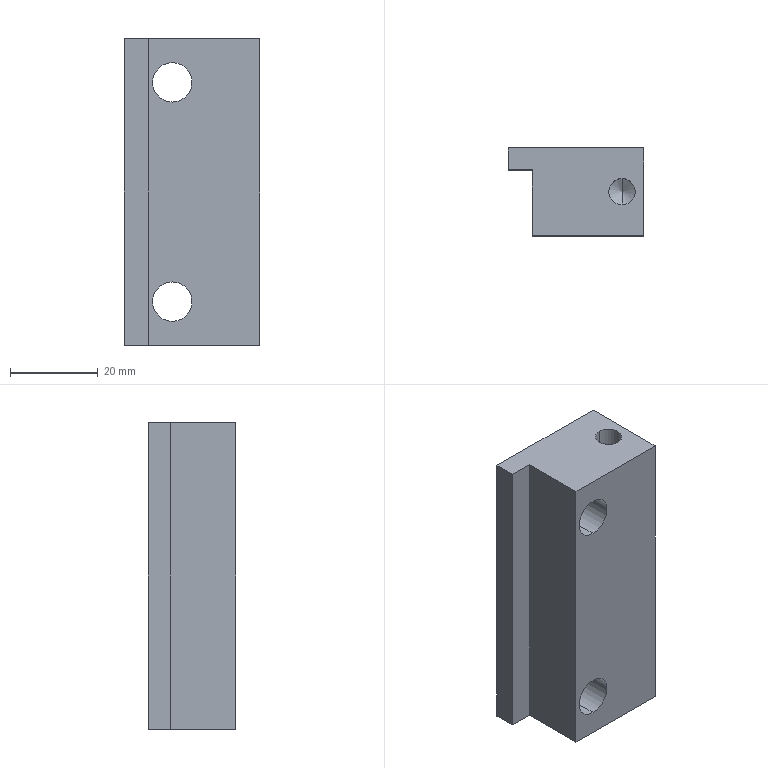Component | SolidWorks | CTM-T-12-AG-05-1 | 1 solid | 20 faces | box 31 x 20 x 70 mm | volume 34085 mm3 | cylinder 8 | plane 8 | cone 4 | commonest cylinder face diameters 9 x4 6 x4 | material Q235A
build123d program:
from build123d import *

# Parameters (mm, degrees)
BOSS_EXTRUDE1_DEPTH      = 70
M6_TAPPED_HOLE1_D        = 6
M6_TAPPED_HOLE1_DEPTH    = 17
M6_TAPPED_HOLE1_TIP      = 1.803
M6_TAPPED_HOLE2_D        = 6
M6_TAPPED_HOLE2_DEPTH    = 17
M6_TAPPED_HOLE2_TIP      = 1.803
M8_CLEARANCE_HOLE1_D     = 9
M8_CLEARANCE_HOLE1_DEPTH = 20
M8_CLEARANCE_HOLE1_TIP   = 2.704


with BuildPart() as part:
    # Sketch1 → Boss-Extrude1 (new body)
    with BuildSketch(Plane.XY):
        Polygon((5, 31), (5, 25.5), (20, 25.5), (20, 0), (0, 0), (0, 31), align=None)
    extrude(amount=BOSS_EXTRUDE1_DEPTH)

    # M6 Tapped Hole1
    with Locations(Plane(origin=(0, 0, 0), x_dir=(-1, 0, 0), z_dir=(0, 0, -1))):
        with Locations((-10, 5)):
            Hole(M6_TAPPED_HOLE1_D / 2, depth=M6_TAPPED_HOLE1_DEPTH)
            with Locations((0, 0, -(M6_TAPPED_HOLE1_DEPTH + M6_TAPPED_HOLE1_TIP / 2))):  # 118° drill point
                Cone(0, M6_TAPPED_HOLE1_D / 2, M6_TAPPED_HOLE1_TIP, mode=Mode.SUBTRACT)

    # M6 Tapped Hole2
    with Locations(Plane.XY.offset(70)):
        with Locations((10, 5)):
            Hole(M6_TAPPED_HOLE2_D / 2, depth=M6_TAPPED_HOLE2_DEPTH)
            with Locations((0, 0, -(M6_TAPPED_HOLE2_DEPTH + M6_TAPPED_HOLE2_TIP / 2))):  # 118° drill point
                Cone(0, M6_TAPPED_HOLE2_D / 2, M6_TAPPED_HOLE2_TIP, mode=Mode.SUBTRACT)

    # M8 Clearance Hole1
    with Locations(Plane.ZY):
        with Locations((10, 20), (60, 20)):
            Hole(M8_CLEARANCE_HOLE1_D / 2, depth=M8_CLEARANCE_HOLE1_DEPTH)
            with Locations((0, 0, -(M8_CLEARANCE_HOLE1_DEPTH + M8_CLEARANCE_HOLE1_TIP / 2))):  # 118° drill point
                Cone(0, M8_CLEARANCE_HOLE1_D / 2, M8_CLEARANCE_HOLE1_TIP, mode=Mode.SUBTRACT)


solid = part.part

# Placed as in the assembly
solid = solid.moved(Location((90.4, 0, 70), (180, 0, 90)))
STEP:
#1=CARTESIAN_POINT('',(2.772,-0.7874,2.539));
#2=VERTEX_POINT('',#1);
#3=CARTESIAN_POINT('',(2.772,-0.7874,2.185));
#4=VERTEX_POINT('',#3);
#5=CARTESIAN_POINT('',(2.772,-0.7874,2.362));
#6=DIRECTION('',(0.,1.,0.));
#7=DIRECTION('',(0.,0.,-1.));
#8=AXIS2_PLACEMENT_3D('',#5,#6,#7);
#9=CIRCLE('',#8,0.1772);
#10=EDGE_CURVE('',#2,#4,#9,.T.);
#11=ORIENTED_EDGE('',*,*,#10,.F.);
#12=CARTESIAN_POINT('',(2.772,0.,2.539));
#13=VERTEX_POINT('',#12);
#14=CARTESIAN_POINT('',(2.772,0.,2.539));
#15=DIRECTION('',(0.,1.,0.));
#16=VECTOR('',#15,39.37);
#17=LINE('',#14,#16);
#18=EDGE_CURVE('',#2,#13,#17,.T.);
#19=ORIENTED_EDGE('',*,*,#18,.T.);
#20=CARTESIAN_POINT('',(2.772,0.,2.185));
#21=VERTEX_POINT('',#20);
#22=CARTESIAN_POINT('',(2.772,0.,2.362));
#23=DIRECTION('',(0.,1.,0.));
#24=DIRECTION('',(0.,0.,-1.));
#25=AXIS2_PLACEMENT_3D('',#22,#23,#24);
#26=CIRCLE('',#25,0.1772);
#27=EDGE_CURVE('',#13,#21,#26,.T.);
#28=ORIENTED_EDGE('',*,*,#27,.T.);
#29=CARTESIAN_POINT('',(2.772,0.,2.185));
#30=DIRECTION('',(0.,1.,0.));
#31=VECTOR('',#30,39.37);
#32=LINE('',#29,#31);
#33=EDGE_CURVE('',#4,#21,#32,.T.);
#34=ORIENTED_EDGE('',*,*,#33,.F.);
#35=EDGE_LOOP('',(#11,#19,#28,#34));
#36=FACE_OUTER_BOUND('',#35,.T.);
#37=CARTESIAN_POINT('',(2.772,0.,2.362));
#38=DIRECTION('',(0.,1.,0.));
#39=DIRECTION('',(0.,0.,-1.));
#40=AXIS2_PLACEMENT_3D('',#37,#38,#39);
#41=CYLINDRICAL_SURFACE('',#40,0.1772);
#42=ADVANCED_FACE('',(#36),#41,.F.);
#43=CARTESIAN_POINT('',(2.772,-0.7874,0.5709));
#44=VERTEX_POINT('',#43);
#45=CARTESIAN_POINT('',(2.772,-0.7874,0.2165));
#46=VERTEX_POINT('',#45);
#47=CARTESIAN_POINT('',(2.772,-0.7874,0.3937));
#48=DIRECTION('',(0.,1.,0.));
#49=DIRECTION('',(0.,0.,-1.));
#50=AXIS2_PLACEMENT_3D('',#47,#48,#49);
#51=CIRCLE('',#50,0.1772);
#52=EDGE_CURVE('',#44,#46,#51,.T.);
#53=ORIENTED_EDGE('',*,*,#52,.F.);
#54=CARTESIAN_POINT('',(2.772,0.,0.5709));
#55=VERTEX_POINT('',#54);
#56=CARTESIAN_POINT('',(2.772,0.,0.5709));
#57=DIRECTION('',(0.,1.,0.));
#58=VECTOR('',#57,39.37);
#59=LINE('',#56,#58);
#60=EDGE_CURVE('',#44,#55,#59,.T.);
#61=ORIENTED_EDGE('',*,*,#60,.T.);
#62=CARTESIAN_POINT('',(2.772,0.,0.2165));
#63=VERTEX_POINT('',#62);
#64=CARTESIAN_POINT('',(2.772,0.,0.3937));
#65=DIRECTION('',(0.,1.,0.));
#66=DIRECTION('',(0.,0.,-1.));
#67=AXIS2_PLACEMENT_3D('',#64,#65,#66);
#68=CIRCLE('',#67,0.1772);
#69=EDGE_CURVE('',#55,#63,#68,.T.);
#70=ORIENTED_EDGE('',*,*,#69,.T.);
#71=CARTESIAN_POINT('',(2.772,0.,0.2165));
#72=DIRECTION('',(0.,1.,0.));
#73=VECTOR('',#72,39.37);
#74=LINE('',#71,#73);
#75=EDGE_CURVE('',#46,#63,#74,.T.);
#76=ORIENTED_EDGE('',*,*,#75,.F.);
#77=EDGE_LOOP('',(#53,#61,#70,#76));
#78=FACE_OUTER_BOUND('',#77,.T.);
#79=CARTESIAN_POINT('',(2.772,0.,0.3937));
#80=DIRECTION('',(0.,1.,0.));
#81=DIRECTION('',(0.,0.,-1.));
#82=AXIS2_PLACEMENT_3D('',#79,#80,#81);
#83=CYLINDRICAL_SURFACE('',#82,0.1772);
#84=ADVANCED_FACE('',(#78),#83,.F.);
#85=CARTESIAN_POINT('',(3.362,-0.2756,0.6693));
#86=VERTEX_POINT('',#85);
#87=CARTESIAN_POINT('',(3.362,-0.5118,0.6693));
#88=VERTEX_POINT('',#87);
#89=CARTESIAN_POINT('',(3.362,-0.3937,0.6693));
#90=DIRECTION('',(0.,0.,-1.));
#91=DIRECTION('',(0.,-1.,0.));
#92=AXIS2_PLACEMENT_3D('',#89,#90,#91);
#93=CIRCLE('',#92,0.1181);
#94=EDGE_CURVE('',#86,#88,#93,.T.);
#95=ORIENTED_EDGE('',*,*,#94,.F.);
#96=CARTESIAN_POINT('',(3.362,-0.2756,-0.));
#97=VERTEX_POINT('',#96);
#98=CARTESIAN_POINT('',(3.362,-0.2756,-0.));
#99=DIRECTION('',(0.,0.,-1.));
#100=VECTOR('',#99,39.37);
#101=LINE('',#98,#100);
#102=EDGE_CURVE('',#86,#97,#101,.T.);
#103=ORIENTED_EDGE('',*,*,#102,.T.);
#104=CARTESIAN_POINT('',(3.362,-0.5118,-0.));
#105=VERTEX_POINT('',#104);
#106=CARTESIAN_POINT('',(3.362,-0.3937,-0.));
#107=DIRECTION('',(0.,0.,-1.));
#108=DIRECTION('',(0.,-1.,-0.));
#109=AXIS2_PLACEMENT_3D('',#106,#107,#108);
#110=CIRCLE('',#109,0.1181);
#111=EDGE_CURVE('',#97,#105,#110,.T.);
#112=ORIENTED_EDGE('',*,*,#111,.T.);
#113=CARTESIAN_POINT('',(3.362,-0.5118,-0.));
#114=DIRECTION('',(0.,0.,-1.));
#115=VECTOR('',#114,39.37);
#116=LINE('',#113,#115);
#117=EDGE_CURVE('',#88,#105,#116,.T.);
#118=ORIENTED_EDGE('',*,*,#117,.F.);
#119=EDGE_LOOP('',(#95,#103,#112,#118));
#120=FACE_OUTER_BOUND('',#119,.T.);
#121=CARTESIAN_POINT('',(3.362,-0.3937,-0.));
#122=DIRECTION('',(0.,0.,-1.));
#123=DIRECTION('',(0.,-1.,-0.));
#124=AXIS2_PLACEMENT_3D('',#121,#122,#123);
#125=CYLINDRICAL_SURFACE('',#124,0.1181);
#126=ADVANCED_FACE('',(#120),#125,.F.);
#127=CARTESIAN_POINT('',(3.362,-0.3937,0.7403));
#128=VERTEX_POINT('',#127);
#129=CARTESIAN_POINT('',(3.362,-0.5118,0.6693));
#130=DIRECTION('',(-0.,-0.8572,-0.515));
#131=VECTOR('',#130,39.37);
#132=LINE('',#129,#131);
#133=EDGE_CURVE('',#128,#88,#132,.T.);
#134=ORIENTED_EDGE('',*,*,#133,.F.);
#135=CARTESIAN_POINT('',(3.362,-0.2756,0.6693));
#136=DIRECTION('',(0.,0.8572,-0.515));
#137=VECTOR('',#136,39.37);
#138=LINE('',#135,#137);
#139=EDGE_CURVE('',#128,#86,#138,.T.);
#140=ORIENTED_EDGE('',*,*,#139,.T.);
#141=ORIENTED_EDGE('',*,*,#94,.T.);
#142=EDGE_LOOP('',(#134,#140,#141));
#143=FACE_OUTER_BOUND('',#142,.T.);
#144=CARTESIAN_POINT('',(3.362,-0.3937,0.6693));
#145=DIRECTION('',(0.,0.,-1.));
#146=DIRECTION('',(0.,-1.,0.));
#147=AXIS2_PLACEMENT_3D('',#144,#145,#146);
#148=CONICAL_SURFACE('',#147,0.1181,1.03);
#149=ADVANCED_FACE('',(#143),#148,.F.);
#150=CARTESIAN_POINT('',(3.362,-0.5118,2.087));
#151=VERTEX_POINT('',#150);
#152=CARTESIAN_POINT('',(3.362,-0.2756,2.087));
#153=VERTEX_POINT('',#152);
#154=CARTESIAN_POINT('',(3.362,-0.3937,2.087));
#155=DIRECTION('',(-0.,-0.,1.));
#156=DIRECTION('',(0.,1.,0.));
#157=AXIS2_PLACEMENT_3D('',#154,#155,#156);
#158=CIRCLE('',#157,0.1181);
#159=EDGE_CURVE('',#151,#153,#158,.T.);
#160=ORIENTED_EDGE('',*,*,#159,.F.);
#161=CARTESIAN_POINT('',(3.362,-0.5118,2.756));
#162=VERTEX_POINT('',#161);
#163=CARTESIAN_POINT('',(3.362,-0.5118,2.756));
#164=DIRECTION('',(-0.,-0.,1.));
#165=VECTOR('',#164,39.37);
#166=LINE('',#163,#165);
#167=EDGE_CURVE('',#151,#162,#166,.T.);
#168=ORIENTED_EDGE('',*,*,#167,.T.);
#169=CARTESIAN_POINT('',(3.362,-0.2756,2.756));
#170=VERTEX_POINT('',#169);
#171=CARTESIAN_POINT('',(3.362,-0.3937,2.756));
#172=DIRECTION('',(-0.,-0.,1.));
#173=DIRECTION('',(0.,1.,0.));
#174=AXIS2_PLACEMENT_3D('',#171,#172,#173);
#175=CIRCLE('',#174,0.1181);
#176=EDGE_CURVE('',#162,#170,#175,.T.);
#177=ORIENTED_EDGE('',*,*,#176,.T.);
#178=CARTESIAN_POINT('',(3.362,-0.2756,2.756));
#179=DIRECTION('',(-0.,-0.,1.));
#180=VECTOR('',#179,39.37);
#181=LINE('',#178,#180);
#182=EDGE_CURVE('',#153,#170,#181,.T.);
#183=ORIENTED_EDGE('',*,*,#182,.F.);
#184=EDGE_LOOP('',(#160,#168,#177,#183));
#185=FACE_OUTER_BOUND('',#184,.T.);
#186=CARTESIAN_POINT('',(3.362,-0.3937,2.756));
#187=DIRECTION('',(-0.,-0.,1.));
#188=DIRECTION('',(0.,1.,0.));
#189=AXIS2_PLACEMENT_3D('',#186,#187,#188);
#190=CYLINDRICAL_SURFACE('',#189,0.1181);
#191=ADVANCED_FACE('',(#185),#190,.F.);
#192=CARTESIAN_POINT('',(3.362,-0.3937,2.016));
#193=VERTEX_POINT('',#192);
#194=CARTESIAN_POINT('',(3.362,-0.2756,2.087));
#195=DIRECTION('',(0.,0.8572,0.515));
#196=VECTOR('',#195,39.37);
#197=LINE('',#194,#196);
#198=EDGE_CURVE('',#193,#153,#197,.T.);
#199=ORIENTED_EDGE('',*,*,#198,.F.);
#200=CARTESIAN_POINT('',(3.362,-0.5118,2.087));
#201=DIRECTION('',(-0.,-0.8572,0.515));
#202=VECTOR('',#201,39.37);
#203=LINE('',#200,#202);
#204=EDGE_CURVE('',#193,#151,#203,.T.);
#205=ORIENTED_EDGE('',*,*,#204,.T.);
#206=ORIENTED_EDGE('',*,*,#159,.T.);
#207=EDGE_LOOP('',(#199,#205,#206));
#208=FACE_OUTER_BOUND('',#207,.T.);
#209=CARTESIAN_POINT('',(3.362,-0.3937,2.087));
#210=DIRECTION('',(-0.,-0.,1.));
#211=DIRECTION('',(0.,1.,0.));
#212=AXIS2_PLACEMENT_3D('',#209,#210,#211);
#213=CONICAL_SURFACE('',#212,0.1181,1.03);
#214=ADVANCED_FACE('',(#208),#213,.F.);
#215=CARTESIAN_POINT('',(2.772,0.,2.362));
#216=DIRECTION('',(0.,1.,0.));
#217=DIRECTION('',(0.,0.,-1.));
#218=AXIS2_PLACEMENT_3D('',#215,#216,#217);
#219=CIRCLE('',#218,0.1772);
#220=EDGE_CURVE('',#21,#13,#219,.T.);
#221=ORIENTED_EDGE('',*,*,#220,.F.);
#222=ORIENTED_EDGE('',*,*,#27,.F.);
#223=EDGE_LOOP('',(#221,#222));
#224=FACE_BOUND('',#223,.T.);
#225=CARTESIAN_POINT('',(2.772,0.,0.3937));
#226=DIRECTION('',(0.,1.,0.));
#227=DIRECTION('',(0.,0.,-1.));
#228=AXIS2_PLACEMENT_3D('',#225,#226,#227);
#229=CIRCLE('',#228,0.1772);
#230=EDGE_CURVE('',#63,#55,#229,.T.);
#231=ORIENTED_EDGE('',*,*,#230,.F.);
#232=ORIENTED_EDGE('',*,*,#69,.F.);
#233=EDGE_LOOP('',(#231,#232));
#234=FACE_BOUND('',#233,.T.);
#235=CARTESIAN_POINT('',(2.339,0.,2.756));
#236=VERTEX_POINT('',#235);
#237=CARTESIAN_POINT('',(3.559,0.,2.756));
#238=VERTEX_POINT('',#237);
#239=CARTESIAN_POINT('',(3.559,0.,2.756));
#240=DIRECTION('',(1.,-0.,0.));
#241=VECTOR('',#240,39.37);
#242=LINE('',#239,#241);
#243=EDGE_CURVE('',#236,#238,#242,.T.);
#244=ORIENTED_EDGE('',*,*,#243,.T.);
#245=CARTESIAN_POINT('',(3.559,0.,-0.));
#246=VERTEX_POINT('',#245);
#247=CARTESIAN_POINT('',(3.559,0.,-0.));
#248=DIRECTION('',(-0.,-0.,1.));
#249=VECTOR('',#248,39.37);
#250=LINE('',#247,#249);
#251=EDGE_CURVE('',#246,#238,#250,.T.);
#252=ORIENTED_EDGE('',*,*,#251,.F.);
#253=CARTESIAN_POINT('',(2.339,0.,-0.));
#254=VERTEX_POINT('',#253);
#255=CARTESIAN_POINT('',(3.559,0.,-0.));
#256=DIRECTION('',(1.,-0.,0.));
#257=VECTOR('',#256,39.37);
#258=LINE('',#255,#257);
#259=EDGE_CURVE('',#254,#246,#258,.T.);
#260=ORIENTED_EDGE('',*,*,#259,.F.);
#261=CARTESIAN_POINT('',(2.339,0.,-0.));
#262=DIRECTION('',(-0.,-0.,1.));
#263=VECTOR('',#262,39.37);
#264=LINE('',#261,#263);
#265=EDGE_CURVE('',#254,#236,#264,.T.);
#266=ORIENTED_EDGE('',*,*,#265,.T.);
#267=EDGE_LOOP('',(#244,#252,#260,#266));
#268=FACE_OUTER_BOUND('',#267,.T.);
#269=CARTESIAN_POINT('',(3.559,0.,-0.));
#270=DIRECTION('',(-0.,-1.,-0.));
#271=DIRECTION('',(-0.,-0.,1.));
#272=AXIS2_PLACEMENT_3D('',#269,#270,#271);
#273=PLANE('',#272);
#274=ADVANCED_FACE('',(#224,#234,#268),#273,.F.);
#275=CARTESIAN_POINT('',(3.559,-0.7874,2.756));
#276=VERTEX_POINT('',#275);
#277=CARTESIAN_POINT('',(3.559,0.,2.756));
#278=DIRECTION('',(-0.,-1.,-0.));
#279=VECTOR('',#278,39.37);
#280=LINE('',#277,#279);
#281=EDGE_CURVE('',#238,#276,#280,.T.);
#282=ORIENTED_EDGE('',*,*,#281,.T.);
#283=CARTESIAN_POINT('',(3.559,-0.7874,-0.));
#284=VERTEX_POINT('',#283);
#285=CARTESIAN_POINT('',(3.559,-0.7874,-0.));
#286=DIRECTION('',(-0.,-0.,1.));
#287=VECTOR('',#286,39.37);
#288=LINE('',#285,#287);
#289=EDGE_CURVE('',#284,#276,#288,.T.);
#290=ORIENTED_EDGE('',*,*,#289,.F.);
#291=CARTESIAN_POINT('',(3.559,0.,-0.));
#292=DIRECTION('',(-0.,-1.,-0.));
#293=VECTOR('',#292,39.37);
#294=LINE('',#291,#293);
#295=EDGE_CURVE('',#246,#284,#294,.T.);
#296=ORIENTED_EDGE('',*,*,#295,.F.);
#297=ORIENTED_EDGE('',*,*,#251,.T.);
#298=EDGE_LOOP('',(#282,#290,#296,#297));
#299=FACE_OUTER_BOUND('',#298,.T.);
#300=CARTESIAN_POINT('',(3.559,0.,-0.));
#301=DIRECTION('',(-1.,0.,-0.));
#302=DIRECTION('',(0.,0.,-1.));
#303=AXIS2_PLACEMENT_3D('',#300,#301,#302);
#304=PLANE('',#303);
#305=ADVANCED_FACE('',(#299),#304,.F.);
#306=CARTESIAN_POINT('',(2.772,-0.7874,2.362));
#307=DIRECTION('',(0.,1.,0.));
#308=DIRECTION('',(0.,0.,-1.));
#309=AXIS2_PLACEMENT_3D('',#306,#307,#308);
#310=CIRCLE('',#309,0.1772);
#311=EDGE_CURVE('',#4,#2,#310,.T.);
#312=ORIENTED_EDGE('',*,*,#311,.T.);
#313=ORIENTED_EDGE('',*,*,#10,.T.);
#314=EDGE_LOOP('',(#312,#313));
#315=FACE_BOUND('',#314,.T.);
#316=CARTESIAN_POINT('',(2.772,-0.7874,0.3937));
#317=DIRECTION('',(0.,1.,0.));
#318=DIRECTION('',(0.,0.,-1.));
#319=AXIS2_PLACEMENT_3D('',#316,#317,#318);
#320=CIRCLE('',#319,0.1772);
#321=EDGE_CURVE('',#46,#44,#320,.T.);
#322=ORIENTED_EDGE('',*,*,#321,.T.);
#323=ORIENTED_EDGE('',*,*,#52,.T.);
#324=EDGE_LOOP('',(#322,#323));
#325=FACE_BOUND('',#324,.T.);
#326=CARTESIAN_POINT('',(2.555,-0.7874,2.756));
#327=VERTEX_POINT('',#326);
#328=CARTESIAN_POINT('',(3.559,-0.7874,2.756));
#329=DIRECTION('',(-1.,0.,-0.));
#330=VECTOR('',#329,39.37);
#331=LINE('',#328,#330);
#332=EDGE_CURVE('',#276,#327,#331,.T.);
#333=ORIENTED_EDGE('',*,*,#332,.T.);
#334=CARTESIAN_POINT('',(2.555,-0.7874,-0.));
#335=VERTEX_POINT('',#334);
#336=CARTESIAN_POINT('',(2.555,-0.7874,-0.));
#337=DIRECTION('',(-0.,-0.,1.));
#338=VECTOR('',#337,39.37);
#339=LINE('',#336,#338);
#340=EDGE_CURVE('',#335,#327,#339,.T.);
#341=ORIENTED_EDGE('',*,*,#340,.F.);
#342=CARTESIAN_POINT('',(3.559,-0.7874,-0.));
#343=DIRECTION('',(-1.,0.,-0.));
#344=VECTOR('',#343,39.37);
#345=LINE('',#342,#344);
#346=EDGE_CURVE('',#284,#335,#345,.T.);
#347=ORIENTED_EDGE('',*,*,#346,.F.);
#348=ORIENTED_EDGE('',*,*,#289,.T.);
#349=EDGE_LOOP('',(#333,#341,#347,#348));
#350=FACE_OUTER_BOUND('',#349,.T.);
#351=CARTESIAN_POINT('',(3.559,-0.7874,-0.));
#352=DIRECTION('',(0.,1.,0.));
#353=DIRECTION('',(1.,-0.,0.));
#354=AXIS2_PLACEMENT_3D('',#351,#352,#353);
#355=PLANE('',#354);
#356=ADVANCED_FACE('',(#315,#325,#350),#355,.F.);
#357=CARTESIAN_POINT('',(2.555,-0.1969,2.756));
#358=VERTEX_POINT('',#357);
#359=CARTESIAN_POINT('',(2.555,-0.1969,2.756));
#360=DIRECTION('',(0.,1.,0.));
#361=VECTOR('',#360,39.37);
#362=LINE('',#359,#361);
#363=EDGE_CURVE('',#327,#358,#362,.T.);
#364=ORIENTED_EDGE('',*,*,#363,.T.);
#365=CARTESIAN_POINT('',(2.555,-0.1969,-0.));
#366=VERTEX_POINT('',#365);
#367=CARTESIAN_POINT('',(2.555,-0.1969,-0.));
#368=DIRECTION('',(-0.,-0.,1.));
#369=VECTOR('',#368,39.37);
#370=LINE('',#367,#369);
#371=EDGE_CURVE('',#366,#358,#370,.T.);
#372=ORIENTED_EDGE('',*,*,#371,.F.);
#373=CARTESIAN_POINT('',(2.555,-0.1969,-0.));
#374=DIRECTION('',(0.,1.,0.));
#375=VECTOR('',#374,39.37);
#376=LINE('',#373,#375);
#377=EDGE_CURVE('',#335,#366,#376,.T.);
#378=ORIENTED_EDGE('',*,*,#377,.F.);
#379=ORIENTED_EDGE('',*,*,#340,.T.);
#380=EDGE_LOOP('',(#364,#372,#378,#379));
#381=FACE_OUTER_BOUND('',#380,.T.);
#382=CARTESIAN_POINT('',(2.555,-0.1969,-0.));
#383=DIRECTION('',(1.,-0.,0.));
#384=DIRECTION('',(-0.,-0.,1.));
#385=AXIS2_PLACEMENT_3D('',#382,#383,#384);
#386=PLANE('',#385);
#387=ADVANCED_FACE('',(#381),#386,.F.);
#388=CARTESIAN_POINT('',(2.339,-0.1969,2.756));
#389=VERTEX_POINT('',#388);
#390=CARTESIAN_POINT('',(2.339,-0.1969,2.756));
#391=DIRECTION('',(-1.,0.,-0.));
#392=VECTOR('',#391,39.37);
#393=LINE('',#390,#392);
#394=EDGE_CURVE('',#358,#389,#393,.T.);
#395=ORIENTED_EDGE('',*,*,#394,.T.);
#396=CARTESIAN_POINT('',(2.339,-0.1969,-0.));
#397=VERTEX_POINT('',#396);
#398=CARTESIAN_POINT('',(2.339,-0.1969,-0.));
#399=DIRECTION('',(-0.,-0.,1.));
#400=VECTOR('',#399,39.37);
#401=LINE('',#398,#400);
#402=EDGE_CURVE('',#397,#389,#401,.T.);
#403=ORIENTED_EDGE('',*,*,#402,.F.);
#404=CARTESIAN_POINT('',(2.339,-0.1969,-0.));
#405=DIRECTION('',(-1.,0.,-0.));
#406=VECTOR('',#405,39.37);
#407=LINE('',#404,#406);
#408=EDGE_CURVE('',#366,#397,#407,.T.);
#409=ORIENTED_EDGE('',*,*,#408,.F.);
#410=ORIENTED_EDGE('',*,*,#371,.T.);
#411=EDGE_LOOP('',(#395,#403,#409,#410));
#412=FACE_OUTER_BOUND('',#411,.T.);
#413=CARTESIAN_POINT('',(2.339,-0.1969,-0.));
#414=DIRECTION('',(0.,1.,0.));
#415=DIRECTION('',(0.,0.,-1.));
#416=AXIS2_PLACEMENT_3D('',#413,#414,#415);
#417=PLANE('',#416);
#418=ADVANCED_FACE('',(#412),#417,.F.);
#419=CARTESIAN_POINT('',(2.339,0.,2.756));
#420=DIRECTION('',(0.,1.,0.));
#421=VECTOR('',#420,39.37);
#422=LINE('',#419,#421);
#423=EDGE_CURVE('',#389,#236,#422,.T.);
#424=ORIENTED_EDGE('',*,*,#423,.T.);
#425=ORIENTED_EDGE('',*,*,#265,.F.);
#426=CARTESIAN_POINT('',(2.339,0.,-0.));
#427=DIRECTION('',(0.,1.,0.));
#428=VECTOR('',#427,39.37);
#429=LINE('',#426,#428);
#430=EDGE_CURVE('',#397,#254,#429,.T.);
#431=ORIENTED_EDGE('',*,*,#430,.F.);
#432=ORIENTED_EDGE('',*,*,#402,.T.);
#433=EDGE_LOOP('',(#424,#425,#431,#432));
#434=FACE_OUTER_BOUND('',#433,.T.);
#435=CARTESIAN_POINT('',(2.339,0.,-0.));
#436=DIRECTION('',(1.,-0.,0.));
#437=DIRECTION('',(-0.,-0.,1.));
#438=AXIS2_PLACEMENT_3D('',#435,#436,#437);
#439=PLANE('',#438);
#440=ADVANCED_FACE('',(#434),#439,.F.);
#441=CARTESIAN_POINT('',(3.362,-0.3937,-0.));
#442=DIRECTION('',(0.,0.,-1.));
#443=DIRECTION('',(0.,-1.,-0.));
#444=AXIS2_PLACEMENT_3D('',#441,#442,#443);
#445=CIRCLE('',#444,0.1181);
#446=EDGE_CURVE('',#105,#97,#445,.T.);
#447=ORIENTED_EDGE('',*,*,#446,.F.);
#448=ORIENTED_EDGE('',*,*,#111,.F.);
#449=EDGE_LOOP('',(#447,#448));
#450=FACE_BOUND('',#449,.T.);
#451=ORIENTED_EDGE('',*,*,#259,.T.);
#452=ORIENTED_EDGE('',*,*,#295,.T.);
#453=ORIENTED_EDGE('',*,*,#346,.T.);
#454=ORIENTED_EDGE('',*,*,#377,.T.);
#455=ORIENTED_EDGE('',*,*,#408,.T.);
#456=ORIENTED_EDGE('',*,*,#430,.T.);
#457=EDGE_LOOP('',(#451,#452,#453,#454,#455,#456));
#458=FACE_OUTER_BOUND('',#457,.T.);
#459=CARTESIAN_POINT('',(2.339,0.,-0.));
#460=DIRECTION('',(-0.,-0.,1.));
#461=DIRECTION('',(0.,1.,0.));
#462=AXIS2_PLACEMENT_3D('',#459,#460,#461);
#463=PLANE('',#462);
#464=ADVANCED_FACE('',(#450,#458),#463,.F.);
#465=CARTESIAN_POINT('',(3.362,-0.3937,2.756));
#466=DIRECTION('',(-0.,-0.,1.));
#467=DIRECTION('',(0.,1.,0.));
#468=AXIS2_PLACEMENT_3D('',#465,#466,#467);
#469=CIRCLE('',#468,0.1181);
#470=EDGE_CURVE('',#170,#162,#469,.T.);
#471=ORIENTED_EDGE('',*,*,#470,.F.);
#472=ORIENTED_EDGE('',*,*,#176,.F.);
#473=EDGE_LOOP('',(#471,#472));
#474=FACE_BOUND('',#473,.T.);
#475=ORIENTED_EDGE('',*,*,#243,.F.);
#476=ORIENTED_EDGE('',*,*,#423,.F.);
#477=ORIENTED_EDGE('',*,*,#394,.F.);
#478=ORIENTED_EDGE('',*,*,#363,.F.);
#479=ORIENTED_EDGE('',*,*,#332,.F.);
#480=ORIENTED_EDGE('',*,*,#281,.F.);
#481=EDGE_LOOP('',(#475,#476,#477,#478,#479,#480));
#482=FACE_OUTER_BOUND('',#481,.T.);
#483=CARTESIAN_POINT('',(2.339,0.,2.756));
#484=DIRECTION('',(-0.,-0.,1.));
#485=DIRECTION('',(0.,1.,0.));
#486=AXIS2_PLACEMENT_3D('',#483,#484,#485);
#487=PLANE('',#486);
#488=ADVANCED_FACE('',(#474,#482),#487,.T.);
#489=ORIENTED_EDGE('',*,*,#204,.F.);
#490=ORIENTED_EDGE('',*,*,#198,.T.);
#491=CARTESIAN_POINT('',(3.362,-0.3937,2.087));
#492=DIRECTION('',(-0.,-0.,1.));
#493=DIRECTION('',(0.,1.,0.));
#494=AXIS2_PLACEMENT_3D('',#491,#492,#493);
#495=CIRCLE('',#494,0.1181);
#496=EDGE_CURVE('',#153,#151,#495,.T.);
#497=ORIENTED_EDGE('',*,*,#496,.T.);
#498=EDGE_LOOP('',(#489,#490,#497));
#499=FACE_OUTER_BOUND('',#498,.T.);
#500=CARTESIAN_POINT('',(3.362,-0.3937,2.087));
#501=DIRECTION('',(-0.,-0.,1.));
#502=DIRECTION('',(0.,1.,0.));
#503=AXIS2_PLACEMENT_3D('',#500,#501,#502);
#504=CONICAL_SURFACE('',#503,0.1181,1.03);
#505=ADVANCED_FACE('',(#499),#504,.F.);
#506=ORIENTED_EDGE('',*,*,#167,.F.);
#507=ORIENTED_EDGE('',*,*,#496,.F.);
#508=ORIENTED_EDGE('',*,*,#182,.T.);
#509=ORIENTED_EDGE('',*,*,#470,.T.);
#510=EDGE_LOOP('',(#506,#507,#508,#509));
#511=FACE_OUTER_BOUND('',#510,.T.);
#512=CARTESIAN_POINT('',(3.362,-0.3937,2.756));
#513=DIRECTION('',(-0.,-0.,1.));
#514=DIRECTION('',(0.,1.,0.));
#515=AXIS2_PLACEMENT_3D('',#512,#513,#514);
#516=CYLINDRICAL_SURFACE('',#515,0.1181);
#517=ADVANCED_FACE('',(#511),#516,.F.);
#518=ORIENTED_EDGE('',*,*,#139,.F.);
#519=ORIENTED_EDGE('',*,*,#133,.T.);
#520=CARTESIAN_POINT('',(3.362,-0.3937,0.6693));
#521=DIRECTION('',(0.,0.,-1.));
#522=DIRECTION('',(0.,-1.,0.));
#523=AXIS2_PLACEMENT_3D('',#520,#521,#522);
#524=CIRCLE('',#523,0.1181);
#525=EDGE_CURVE('',#88,#86,#524,.T.);
#526=ORIENTED_EDGE('',*,*,#525,.T.);
#527=EDGE_LOOP('',(#518,#519,#526));
#528=FACE_OUTER_BOUND('',#527,.T.);
#529=CARTESIAN_POINT('',(3.362,-0.3937,0.6693));
#530=DIRECTION('',(0.,0.,-1.));
#531=DIRECTION('',(0.,-1.,0.));
#532=AXIS2_PLACEMENT_3D('',#529,#530,#531);
#533=CONICAL_SURFACE('',#532,0.1181,1.03);
#534=ADVANCED_FACE('',(#528),#533,.F.);
#535=ORIENTED_EDGE('',*,*,#102,.F.);
#536=ORIENTED_EDGE('',*,*,#525,.F.);
#537=ORIENTED_EDGE('',*,*,#117,.T.);
#538=ORIENTED_EDGE('',*,*,#446,.T.);
#539=EDGE_LOOP('',(#535,#536,#537,#538));
#540=FACE_OUTER_BOUND('',#539,.T.);
#541=CARTESIAN_POINT('',(3.362,-0.3937,-0.));
#542=DIRECTION('',(0.,0.,-1.));
#543=DIRECTION('',(0.,-1.,-0.));
#544=AXIS2_PLACEMENT_3D('',#541,#542,#543);
#545=CYLINDRICAL_SURFACE('',#544,0.1181);
#546=ADVANCED_FACE('',(#540),#545,.F.);
#547=ORIENTED_EDGE('',*,*,#60,.F.);
#548=ORIENTED_EDGE('',*,*,#321,.F.);
#549=ORIENTED_EDGE('',*,*,#75,.T.);
#550=ORIENTED_EDGE('',*,*,#230,.T.);
#551=EDGE_LOOP('',(#547,#548,#549,#550));
#552=FACE_OUTER_BOUND('',#551,.T.);
#553=CARTESIAN_POINT('',(2.772,0.,0.3937));
#554=DIRECTION('',(0.,1.,0.));
#555=DIRECTION('',(0.,0.,-1.));
#556=AXIS2_PLACEMENT_3D('',#553,#554,#555);
#557=CYLINDRICAL_SURFACE('',#556,0.1772);
#558=ADVANCED_FACE('',(#552),#557,.F.);
#559=ORIENTED_EDGE('',*,*,#18,.F.);
#560=ORIENTED_EDGE('',*,*,#311,.F.);
#561=ORIENTED_EDGE('',*,*,#33,.T.);
#562=ORIENTED_EDGE('',*,*,#220,.T.);
#563=EDGE_LOOP('',(#559,#560,#561,#562));
#564=FACE_OUTER_BOUND('',#563,.T.);
#565=CARTESIAN_POINT('',(2.772,0.,2.362));
#566=DIRECTION('',(0.,1.,0.));
#567=DIRECTION('',(0.,0.,-1.));
#568=AXIS2_PLACEMENT_3D('',#565,#566,#567);
#569=CYLINDRICAL_SURFACE('',#568,0.1772);
#570=ADVANCED_FACE('',(#564),#569,.F.);
#571=CLOSED_SHELL('',(#42,#84,#126,#149,#191,#214,#274,#305,#356,#387,#418,#440,#464,#488,#505,#517,#534,#546,#558,#570));
#572=MANIFOLD_SOLID_BREP('',#571);
#573=CARTESIAN_POINT('',(0.,0.,0.));
#574=DIRECTION('',(0.,0.,1.));
#575=DIRECTION('',(1.,0.,0.));
#576=AXIS2_PLACEMENT_3D('',#573,#574,#575);
#577=(LENGTH_UNIT()NAMED_UNIT(*)SI_UNIT($,.METRE.));
#578=LENGTH_MEASURE_WITH_UNIT(LENGTH_MEASURE(0.0254),#577);
#579=DIMENSIONAL_EXPONENTS(1.,0.,0.,0.,0.,0.,0.);
#580=(CONVERSION_BASED_UNIT('',#578)LENGTH_UNIT()NAMED_UNIT(#579));
#581=UNCERTAINTY_MEASURE_WITH_UNIT(LENGTH_MEASURE(0.00001),#580,'','');
#582=(NAMED_UNIT(*)PLANE_ANGLE_UNIT()SI_UNIT($,.RADIAN.));
#583=(NAMED_UNIT(*)SI_UNIT($,.STERADIAN.)SOLID_ANGLE_UNIT());
#584=(GEOMETRIC_REPRESENTATION_CONTEXT(3)GLOBAL_UNCERTAINTY_ASSIGNED_CONTEXT((#581))GLOBAL_UNIT_ASSIGNED_CONTEXT((#580,#582,#583))REPRESENTATION_CONTEXT('',''));
#585=ADVANCED_BREP_SHAPE_REPRESENTATION('',(#572,#576),#584);
#586=COLOUR_RGB('',0.7922,0.8196,0.9333);
#587=FILL_AREA_STYLE_COLOUR('',#586);
#588=FILL_AREA_STYLE('',(#587));
#589=SURFACE_STYLE_FILL_AREA(#588);
#590=SURFACE_SIDE_STYLE('',(#589));
#591=SURFACE_STYLE_USAGE(.BOTH.,#590);
#592=PRESENTATION_STYLE_ASSIGNMENT((#591));
#593=STYLED_ITEM('',(#592),#572);
#594=PRESENTATION_LAYER_ASSIGNMENT('','',(#593));
#595=(LENGTH_UNIT()NAMED_UNIT(*)SI_UNIT($,.METRE.));
#596=LENGTH_MEASURE_WITH_UNIT(LENGTH_MEASURE(0.0254),#595);
#597=DIMENSIONAL_EXPONENTS(1.,0.,0.,0.,0.,0.,0.);
#598=(CONVERSION_BASED_UNIT('',#596)LENGTH_UNIT()NAMED_UNIT(#597));
#599=UNCERTAINTY_MEASURE_WITH_UNIT(LENGTH_MEASURE(0.00001),#598,'','');
#600=(NAMED_UNIT(*)PLANE_ANGLE_UNIT()SI_UNIT($,.RADIAN.));
#601=(NAMED_UNIT(*)SI_UNIT($,.STERADIAN.)SOLID_ANGLE_UNIT());
#602=(GEOMETRIC_REPRESENTATION_CONTEXT(3)GLOBAL_UNCERTAINTY_ASSIGNED_CONTEXT((#599))GLOBAL_UNIT_ASSIGNED_CONTEXT((#598,#600,#601))REPRESENTATION_CONTEXT('',''));
#603=MECHANICAL_DESIGN_GEOMETRIC_PRESENTATION_REPRESENTATION('',(#593),#602);